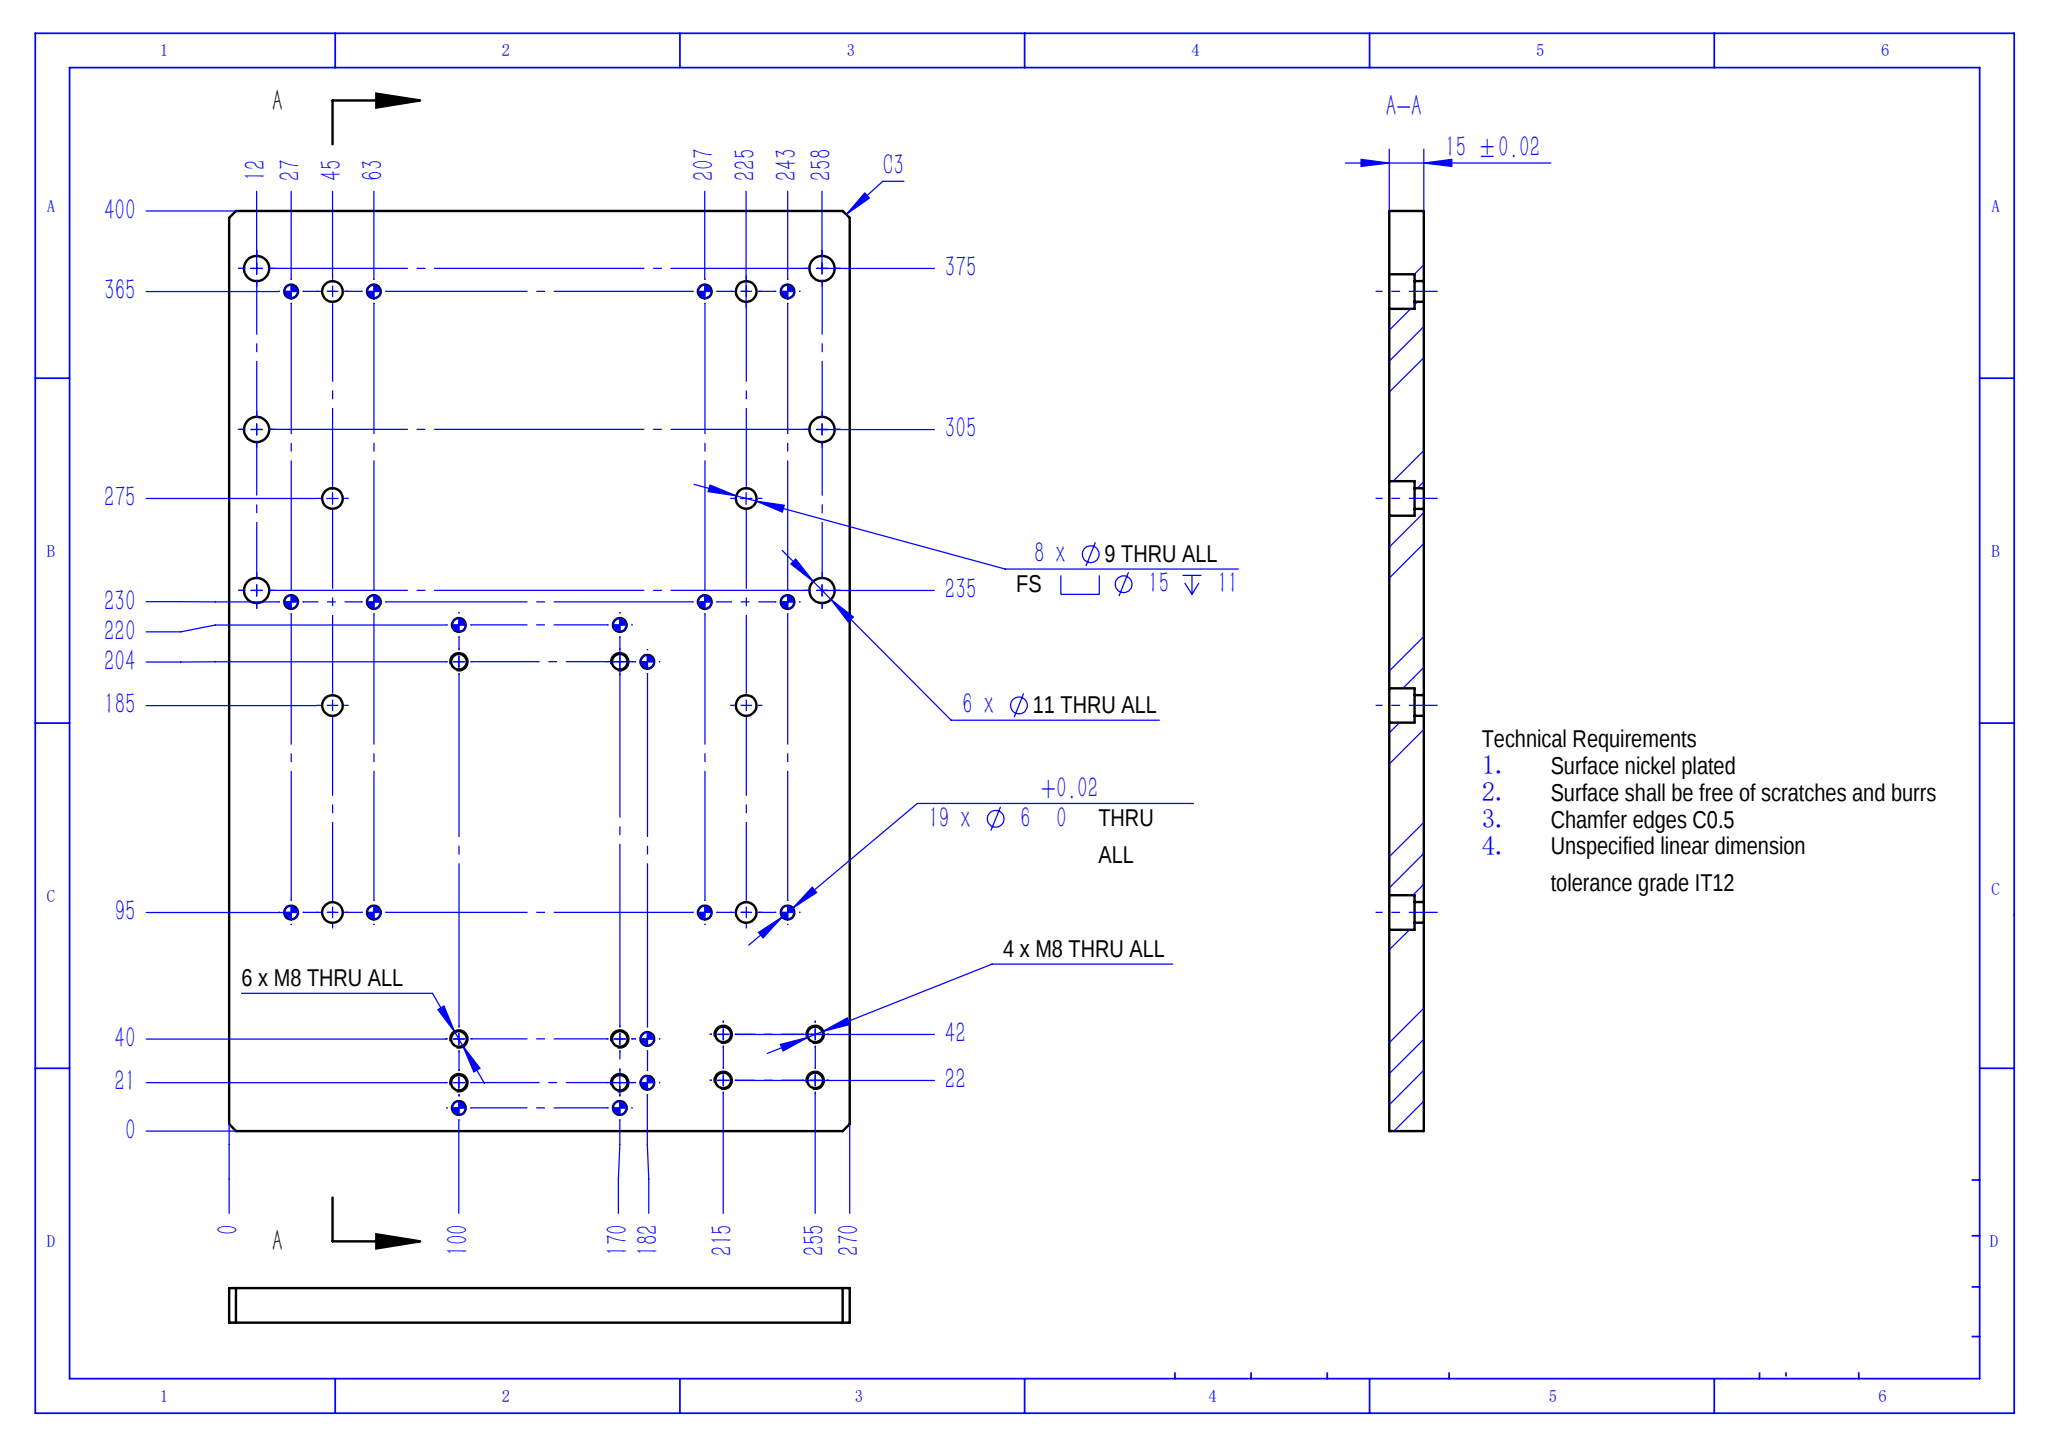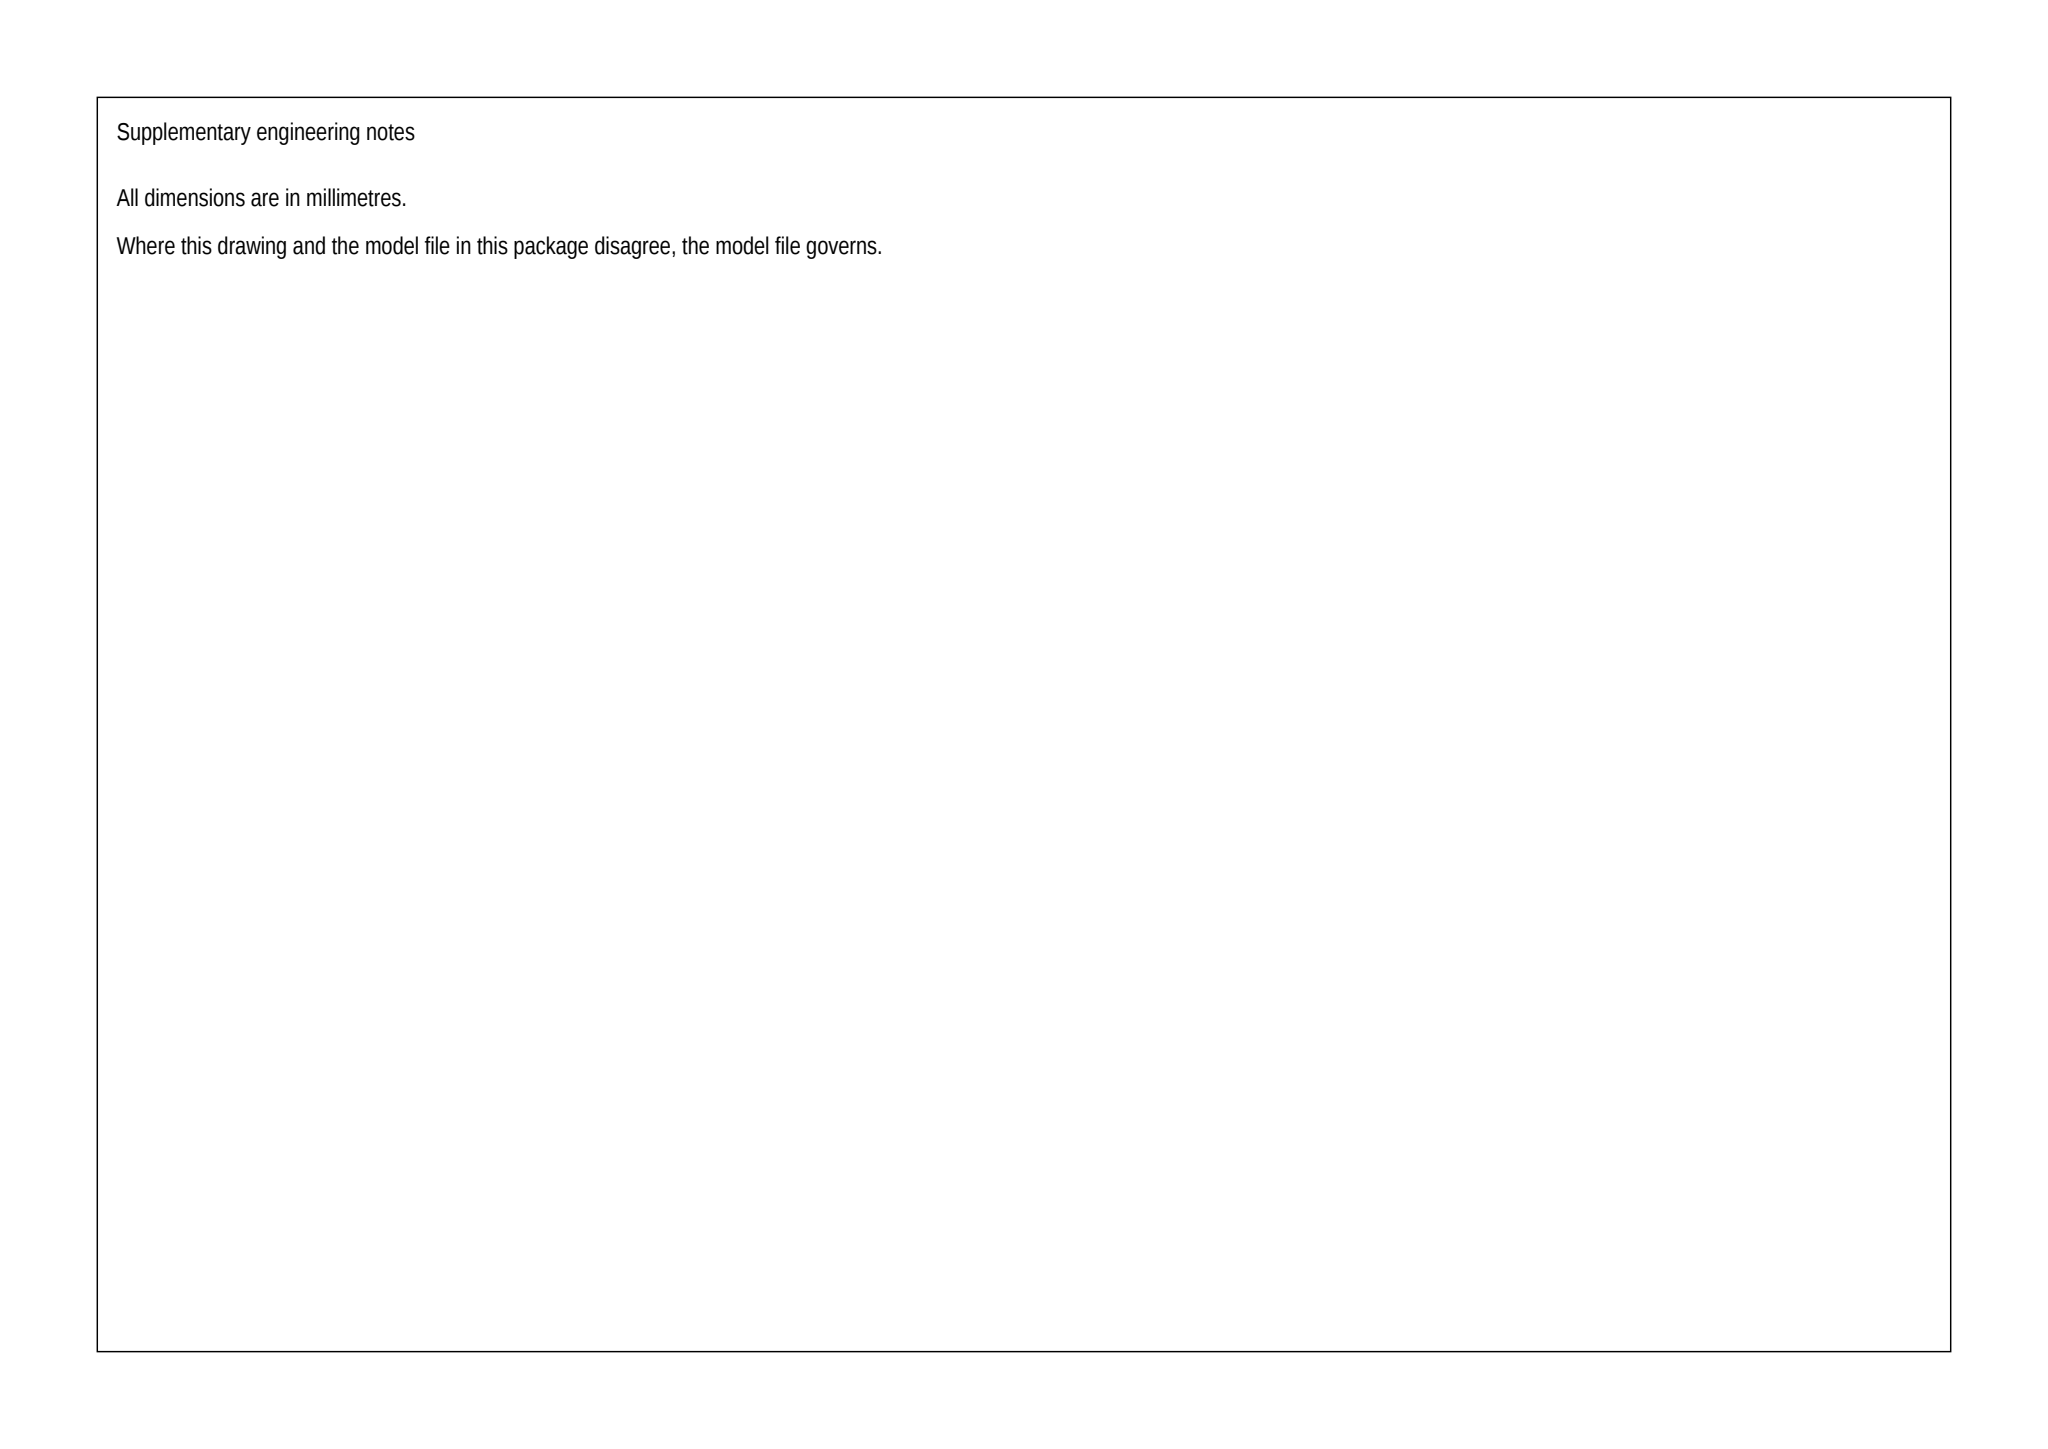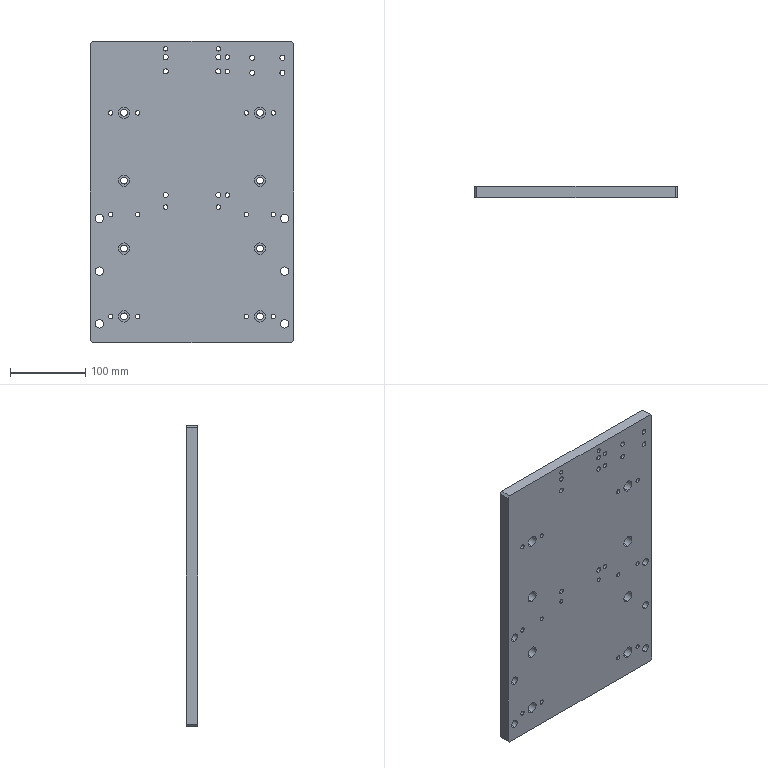Part | SolidWorks | mm | 1 solid | 120 faces | box 270 x 15 x 400 mm | volume 1580085 mm3 | cylinder 102 | plane 18 | commonest cylinder face diameters 6 x38 6.8 x20 15 x16 9 x16 11 x12
build123d program:
from build123d import *

# Parameters (mm, degrees)
SKETCH1_W                                         = 270
SKETCH1_H                                         = 400
BOSS_EXTRUDE1_DEPTH                               = 15
HOLE_SIZE_ACCORDING_TO_TYPE_1_OF_HEXA_D           = 9
HOLE_SIZE_ACCORDING_TO_TYPE_1_OF_HEXA_CBORE_D     = 15
HOLE_SIZE_ACCORDING_TO_TYPE_1_OF_HEXA_CBORE_DEPTH = 11
LPATTERN1_COUNT                                   = 4
LPATTERN1_PITCH                                   = 90
M8_TAPPED_HOLE1_D                                 = 6.8
M10_CLEARANCE_HOLE1_D                             = 11
M8_TAPPED_HOLE2_D                                 = 6.8
CHAMFER1_SIZE                                     = 3
SIZE_MM_DOWEL_PIN_HOLE1_D                         = 6


with BuildPart() as part:
    # Sketch1 → Boss-Extrude1 (new body)
    with BuildSketch(Plane(origin=(0, 0, 0), x_dir=(1, 0, 0), z_dir=(0, 1, 0))):
        Rectangle(SKETCH1_W, SKETCH1_H)
    extrude(amount=BOSS_EXTRUDE1_DEPTH)

    # Hole Size _ according to_ Type 1 of Hexa (through all)
    with Locations(Plane.XZ):
        with Locations((-90, -165), (90, -165)):
            hole_size_according_to_type_1_of_hexa = CounterBoreHole(HOLE_SIZE_ACCORDING_TO_TYPE_1_OF_HEXA_D / 2, HOLE_SIZE_ACCORDING_TO_TYPE_1_OF_HEXA_CBORE_D / 2, HOLE_SIZE_ACCORDING_TO_TYPE_1_OF_HEXA_CBORE_DEPTH)

    # LPattern1: Hole Size _ according to_ Type 1 of Hexa ×4
    with Locations(*[(0, 0, i * LPATTERN1_PITCH) for i in range(1, LPATTERN1_COUNT)]):
        add(hole_size_according_to_type_1_of_hexa, mode=Mode.SUBTRACT)

    # M8 Tapped Hole1 (through all)
    with Locations(Plane(origin=(0, 15, 0), x_dir=(1, 0, 0), z_dir=(0, 1, 0))):
        with Locations((-35, -160), (35, -179), (-35, -179), (35, -160), (-35, 4), (35, 4)):
            Hole(M8_TAPPED_HOLE1_D / 2)

    # M10 Clearance Hole1 (through all)
    with Locations(Plane(origin=(0, 15, 0), x_dir=(1, 0, 0), z_dir=(0, 1, 0))):
        with Locations((-123, 175), (-123, 105), (-123, 35), (123, 35), (123, 175), (123, 105)):
            Hole(M10_CLEARANCE_HOLE1_D / 2)

    # M8 Tapped Hole2 (through all)
    with Locations(Plane(origin=(0, 15, 0), x_dir=(1, 0, 0), z_dir=(0, 1, 0))):
        with Locations((80, -158), (120, -178), (80, -178), (120, -158)):
            Hole(M8_TAPPED_HOLE2_D / 2)

    # Chamfer1
    chamfer1_edges = [part.edges().sort_by_distance(p)[0] for p in [
        (135, 7.5, 200),
        (-135, 7.5, 200),
        (-135, 7.5, -200),
        (135, 7.5, -200),
    ]]
    chamfer(chamfer1_edges, length=CHAMFER1_SIZE)

    # Size mm Dowel Pin Hole1 (through all)
    with Locations(Plane(origin=(0, 15, 0), x_dir=(1, 0, 0), z_dir=(0, 1, 0))):
        with Locations((-108, 165), (-72, -105), (72, 165), (108, -105), (72, -105), (108, 165), (-108, -105), (-72, 165), (108, 30), (72, 30), (-72, 30), (-108, 30), (-35, -190), (35, -190), (-35, 20), (35, 20), (47, -160), (47, -179), (47, 4)):
            Hole(SIZE_MM_DOWEL_PIN_HOLE1_D / 2)


solid = part.part